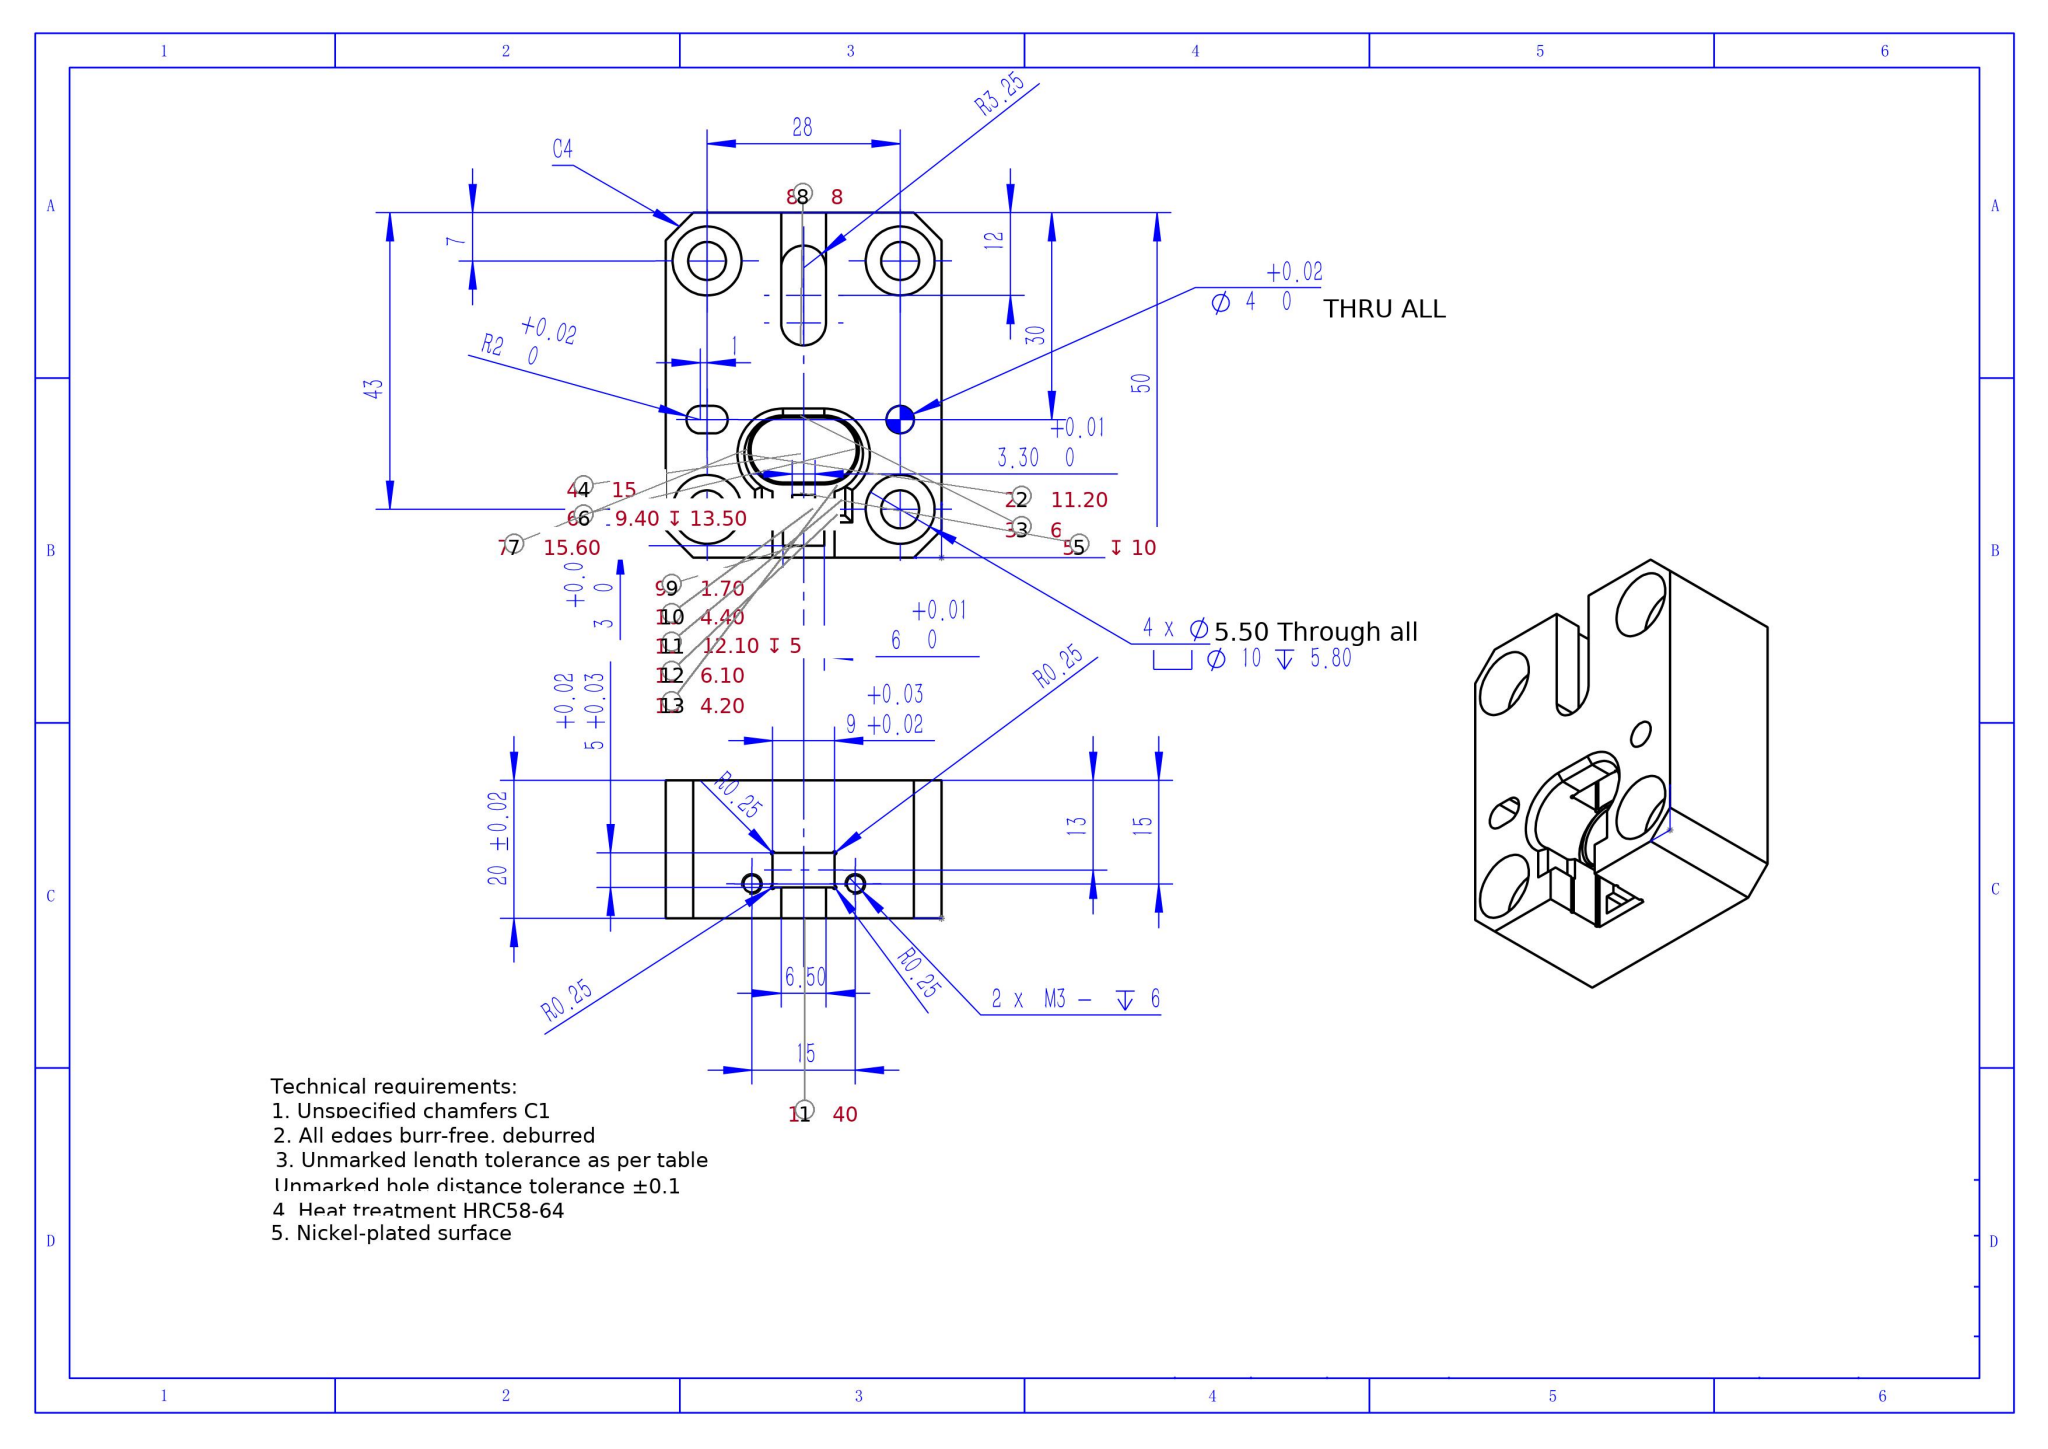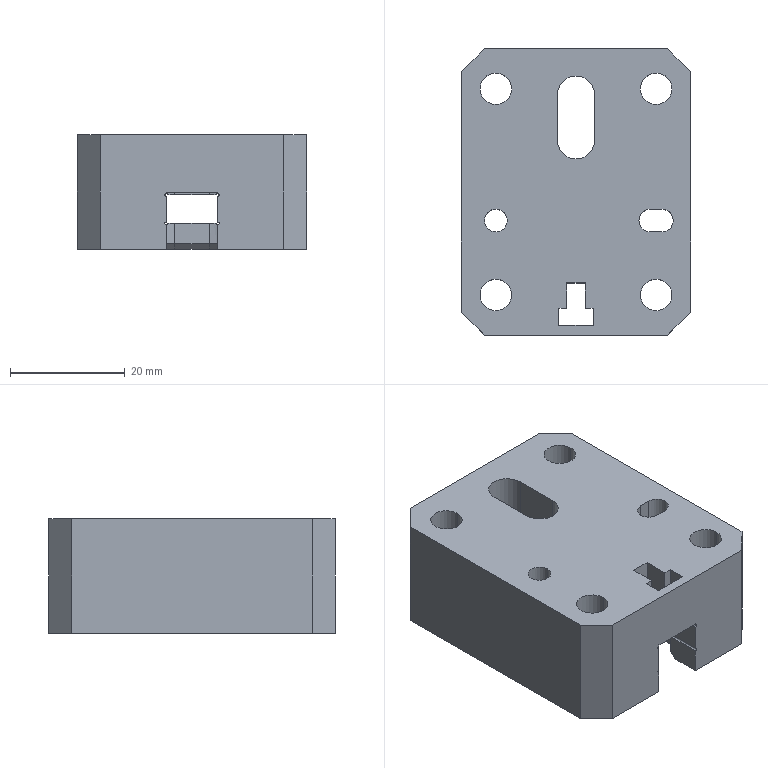Part | SolidWorks | mm | 1 solid | 111 faces | box 40 x 50 x 20 mm | volume 29312 mm3 | plane 57 | cylinder 44 | cone 10 | commonest cylinder face diameters 0.5 x10 10 x8 5.5 x8 4 x5 2.5 x4 9.4 x3 11.2 x3 6.5 x3